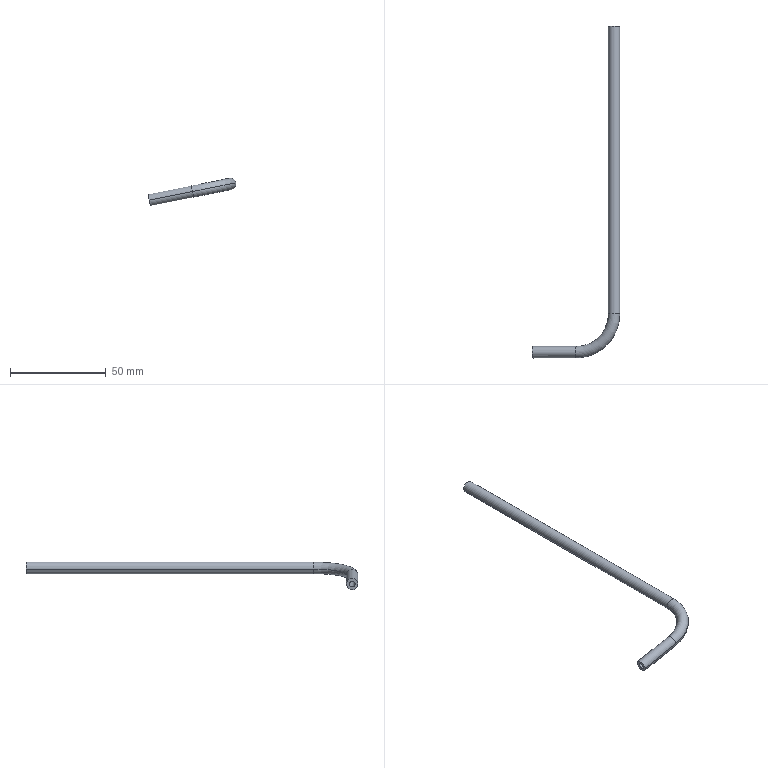Component | SolidWorks | 1-1 | 1 solid | 14 faces | box 45.75 x 173 x 14.39 mm | volume 4335 mm3 | cylinder 8 | torus 4 | plane 2 | commonest cylinder face diameters 3 x4 6 x4
build123d program:
from build123d import *

# Parameters (mm, degrees)
SKETCH7_R   = 3
SKETCH7_R_2 = 1.5


with BuildPart() as part:
    # Sweep2: sweep along a path in Sketch1
    with BuildLine(Plane(origin=(0, 0, 0), x_dir=(1, 0, 0), z_dir=(0, 1, 0))) as sweep2_path:
        Line((0, 0), (0, 23))
        ThreePointArc((0, 23), (-5.858, 37.142), (-20, 43))
        Line((-20, 43), (-170, 43))
    # Sketch7 → Sweep2 (sweep)
    with BuildSketch(Plane(origin=(0, 0, 0), x_dir=(-1, 0, 0), z_dir=(0, 0, -1))):
        Circle(SKETCH7_R)
        Circle(SKETCH7_R_2, mode=Mode.SUBTRACT)
    sweep(path=sweep2_path.line)


solid = part.part

# Placed as in the assembly
solid = solid.moved(Location((80.401, -319.2, 16.115), (-180, -78.666, 90)))
STEP:
#1=CARTESIAN_POINT('',(4.053,-12.508,0.8124));
#2=VERTEX_POINT('',#1);
#3=CARTESIAN_POINT('',(4.053,-12.626,0.8124));
#4=VERTEX_POINT('',#3);
#5=CARTESIAN_POINT('',(4.053,-12.567,0.8124));
#6=DIRECTION('',(-0.9805,-0.,-0.1965));
#7=DIRECTION('',(0.,1.,0.));
#8=AXIS2_PLACEMENT_3D('',#5,#6,#7);
#9=CIRCLE('',#8,0.05906);
#10=EDGE_CURVE('',#2,#4,#9,.T.);
#11=ORIENTED_EDGE('',*,*,#10,.T.);
#12=CARTESIAN_POINT('',(4.883,-11.78,0.9787));
#13=VERTEX_POINT('',#12);
#14=CARTESIAN_POINT('',(4.053,-11.78,0.8124));
#15=DIRECTION('',(-0.1965,-0.,0.9805));
#16=DIRECTION('',(0.9805,0.,0.1965));
#17=AXIS2_PLACEMENT_3D('',#14,#15,#16);
#18=CIRCLE('',#17,0.8465);
#19=EDGE_CURVE('',#4,#13,#18,.T.);
#20=ORIENTED_EDGE('',*,*,#19,.T.);
#21=CARTESIAN_POINT('',(4.767,-11.78,0.9555));
#22=VERTEX_POINT('',#21);
#23=CARTESIAN_POINT('',(4.825,-11.78,0.9671));
#24=DIRECTION('',(0.,-1.,-0.));
#25=DIRECTION('',(-0.9805,0.,-0.1965));
#26=AXIS2_PLACEMENT_3D('',#23,#24,#25);
#27=CIRCLE('',#26,0.05906);
#28=EDGE_CURVE('',#22,#13,#27,.T.);
#29=ORIENTED_EDGE('',*,*,#28,.F.);
#30=CARTESIAN_POINT('',(4.053,-11.78,0.8124));
#31=DIRECTION('',(-0.1965,-0.,0.9805));
#32=DIRECTION('',(0.9805,0.,0.1965));
#33=AXIS2_PLACEMENT_3D('',#30,#31,#32);
#34=CIRCLE('',#33,0.7283);
#35=EDGE_CURVE('',#2,#22,#34,.T.);
#36=ORIENTED_EDGE('',*,*,#35,.F.);
#37=EDGE_LOOP('',(#11,#20,#29,#36));
#38=FACE_OUTER_BOUND('',#37,.T.);
#39=CARTESIAN_POINT('',(4.053,-11.78,0.8124));
#40=DIRECTION('',(-0.1965,-0.,0.9805));
#41=DIRECTION('',(-0.9805,-0.,-0.1965));
#42=AXIS2_PLACEMENT_3D('',#39,#40,#41);
#43=TOROIDAL_SURFACE('',#42,0.7874,0.05906);
#44=ADVANCED_FACE('',(#38),#43,.F.);
#45=CARTESIAN_POINT('',(4.053,-12.449,0.8124));
#46=VERTEX_POINT('',#45);
#47=CARTESIAN_POINT('',(4.053,-12.685,0.8124));
#48=VERTEX_POINT('',#47);
#49=CARTESIAN_POINT('',(4.053,-12.567,0.8124));
#50=DIRECTION('',(0.9805,0.,0.1965));
#51=DIRECTION('',(0.,1.,0.));
#52=AXIS2_PLACEMENT_3D('',#49,#50,#51);
#53=CIRCLE('',#52,0.1181);
#54=EDGE_CURVE('',#46,#48,#53,.T.);
#55=ORIENTED_EDGE('',*,*,#54,.T.);
#56=CARTESIAN_POINT('',(4.941,-11.78,0.9903));
#57=VERTEX_POINT('',#56);
#58=CARTESIAN_POINT('',(4.053,-11.78,0.8124));
#59=DIRECTION('',(-0.1965,-0.,0.9805));
#60=DIRECTION('',(0.9805,0.,0.1965));
#61=AXIS2_PLACEMENT_3D('',#58,#59,#60);
#62=CIRCLE('',#61,0.9055);
#63=EDGE_CURVE('',#48,#57,#62,.T.);
#64=ORIENTED_EDGE('',*,*,#63,.T.);
#65=CARTESIAN_POINT('',(4.709,-11.78,0.9439));
#66=VERTEX_POINT('',#65);
#67=CARTESIAN_POINT('',(4.825,-11.78,0.9671));
#68=DIRECTION('',(-0.,1.,0.));
#69=DIRECTION('',(-0.9805,0.,-0.1965));
#70=AXIS2_PLACEMENT_3D('',#67,#68,#69);
#71=CIRCLE('',#70,0.1181);
#72=EDGE_CURVE('',#66,#57,#71,.T.);
#73=ORIENTED_EDGE('',*,*,#72,.F.);
#74=CARTESIAN_POINT('',(4.053,-11.78,0.8124));
#75=DIRECTION('',(-0.1965,-0.,0.9805));
#76=DIRECTION('',(0.9805,0.,0.1965));
#77=AXIS2_PLACEMENT_3D('',#74,#75,#76);
#78=CIRCLE('',#77,0.6693);
#79=EDGE_CURVE('',#46,#66,#78,.T.);
#80=ORIENTED_EDGE('',*,*,#79,.F.);
#81=EDGE_LOOP('',(#55,#64,#73,#80));
#82=FACE_OUTER_BOUND('',#81,.T.);
#83=CARTESIAN_POINT('',(4.053,-11.78,0.8124));
#84=DIRECTION('',(-0.1965,-0.,0.9805));
#85=DIRECTION('',(-0.9805,0.,-0.1965));
#86=AXIS2_PLACEMENT_3D('',#83,#84,#85);
#87=TOROIDAL_SURFACE('',#86,0.7874,0.1181);
#88=ADVANCED_FACE('',(#82),#87,.T.);
#89=ORIENTED_EDGE('',*,*,#28,.T.);
#90=CARTESIAN_POINT('',(4.883,-5.874,0.9787));
#91=VERTEX_POINT('',#90);
#92=CARTESIAN_POINT('',(4.883,-11.78,0.9787));
#93=DIRECTION('',(-0.,1.,0.));
#94=VECTOR('',#93,39.37);
#95=LINE('',#92,#94);
#96=EDGE_CURVE('',#13,#91,#95,.T.);
#97=ORIENTED_EDGE('',*,*,#96,.T.);
#98=CARTESIAN_POINT('',(4.767,-5.874,0.9555));
#99=VERTEX_POINT('',#98);
#100=CARTESIAN_POINT('',(4.825,-5.874,0.9671));
#101=DIRECTION('',(0.,-1.,-0.));
#102=DIRECTION('',(-0.9805,0.,-0.1965));
#103=AXIS2_PLACEMENT_3D('',#100,#101,#102);
#104=CIRCLE('',#103,0.05906);
#105=EDGE_CURVE('',#99,#91,#104,.T.);
#106=ORIENTED_EDGE('',*,*,#105,.F.);
#107=CARTESIAN_POINT('',(4.767,-11.78,0.9555));
#108=DIRECTION('',(-0.,1.,0.));
#109=VECTOR('',#108,39.37);
#110=LINE('',#107,#109);
#111=EDGE_CURVE('',#22,#99,#110,.T.);
#112=ORIENTED_EDGE('',*,*,#111,.F.);
#113=EDGE_LOOP('',(#89,#97,#106,#112));
#114=FACE_OUTER_BOUND('',#113,.T.);
#115=CARTESIAN_POINT('',(4.825,-11.78,0.9671));
#116=DIRECTION('',(-0.,1.,0.));
#117=DIRECTION('',(-0.9805,0.,-0.1965));
#118=AXIS2_PLACEMENT_3D('',#115,#116,#117);
#119=CYLINDRICAL_SURFACE('',#118,0.05906);
#120=ADVANCED_FACE('',(#114),#119,.F.);
#121=CARTESIAN_POINT('',(3.165,-12.508,0.6344));
#122=VERTEX_POINT('',#121);
#123=CARTESIAN_POINT('',(3.165,-12.626,0.6344));
#124=VERTEX_POINT('',#123);
#125=CARTESIAN_POINT('',(3.165,-12.567,0.6344));
#126=DIRECTION('',(-0.9805,-0.,-0.1965));
#127=DIRECTION('',(0.,1.,0.));
#128=AXIS2_PLACEMENT_3D('',#125,#126,#127);
#129=CIRCLE('',#128,0.05906);
#130=EDGE_CURVE('',#122,#124,#129,.T.);
#131=ORIENTED_EDGE('',*,*,#130,.T.);
#132=CARTESIAN_POINT('',(3.165,-12.626,0.6344));
#133=DIRECTION('',(0.9805,0.,0.1965));
#134=VECTOR('',#133,39.37);
#135=LINE('',#132,#134);
#136=EDGE_CURVE('',#124,#4,#135,.T.);
#137=ORIENTED_EDGE('',*,*,#136,.T.);
#138=ORIENTED_EDGE('',*,*,#10,.F.);
#139=CARTESIAN_POINT('',(3.165,-12.508,0.6344));
#140=DIRECTION('',(0.9805,0.,0.1965));
#141=VECTOR('',#140,39.37);
#142=LINE('',#139,#141);
#143=EDGE_CURVE('',#122,#2,#142,.T.);
#144=ORIENTED_EDGE('',*,*,#143,.F.);
#145=EDGE_LOOP('',(#131,#137,#138,#144));
#146=FACE_OUTER_BOUND('',#145,.T.);
#147=CARTESIAN_POINT('',(3.165,-12.567,0.6344));
#148=DIRECTION('',(0.9805,0.,0.1965));
#149=DIRECTION('',(0.,1.,0.));
#150=AXIS2_PLACEMENT_3D('',#147,#148,#149);
#151=CYLINDRICAL_SURFACE('',#150,0.05906);
#152=ADVANCED_FACE('',(#146),#151,.F.);
#153=ORIENTED_EDGE('',*,*,#72,.T.);
#154=CARTESIAN_POINT('',(4.941,-5.874,0.9903));
#155=VERTEX_POINT('',#154);
#156=CARTESIAN_POINT('',(4.941,-11.78,0.9903));
#157=DIRECTION('',(-0.,1.,0.));
#158=VECTOR('',#157,39.37);
#159=LINE('',#156,#158);
#160=EDGE_CURVE('',#57,#155,#159,.T.);
#161=ORIENTED_EDGE('',*,*,#160,.T.);
#162=CARTESIAN_POINT('',(4.709,-5.874,0.9439));
#163=VERTEX_POINT('',#162);
#164=CARTESIAN_POINT('',(4.825,-5.874,0.9671));
#165=DIRECTION('',(-0.,1.,0.));
#166=DIRECTION('',(-0.9805,0.,-0.1965));
#167=AXIS2_PLACEMENT_3D('',#164,#165,#166);
#168=CIRCLE('',#167,0.1181);
#169=EDGE_CURVE('',#163,#155,#168,.T.);
#170=ORIENTED_EDGE('',*,*,#169,.F.);
#171=CARTESIAN_POINT('',(4.709,-11.78,0.9439));
#172=DIRECTION('',(-0.,1.,0.));
#173=VECTOR('',#172,39.37);
#174=LINE('',#171,#173);
#175=EDGE_CURVE('',#66,#163,#174,.T.);
#176=ORIENTED_EDGE('',*,*,#175,.F.);
#177=EDGE_LOOP('',(#153,#161,#170,#176));
#178=FACE_OUTER_BOUND('',#177,.T.);
#179=CARTESIAN_POINT('',(4.825,-11.78,0.9671));
#180=DIRECTION('',(-0.,1.,0.));
#181=DIRECTION('',(-0.9805,0.,-0.1965));
#182=AXIS2_PLACEMENT_3D('',#179,#180,#181);
#183=CYLINDRICAL_SURFACE('',#182,0.1181);
#184=ADVANCED_FACE('',(#178),#183,.T.);
#185=CARTESIAN_POINT('',(3.165,-12.449,0.6344));
#186=VERTEX_POINT('',#185);
#187=CARTESIAN_POINT('',(3.165,-12.685,0.6344));
#188=VERTEX_POINT('',#187);
#189=CARTESIAN_POINT('',(3.165,-12.567,0.6344));
#190=DIRECTION('',(0.9805,0.,0.1965));
#191=DIRECTION('',(0.,1.,0.));
#192=AXIS2_PLACEMENT_3D('',#189,#190,#191);
#193=CIRCLE('',#192,0.1181);
#194=EDGE_CURVE('',#186,#188,#193,.T.);
#195=ORIENTED_EDGE('',*,*,#194,.T.);
#196=CARTESIAN_POINT('',(3.165,-12.685,0.6344));
#197=DIRECTION('',(0.9805,0.,0.1965));
#198=VECTOR('',#197,39.37);
#199=LINE('',#196,#198);
#200=EDGE_CURVE('',#188,#48,#199,.T.);
#201=ORIENTED_EDGE('',*,*,#200,.T.);
#202=ORIENTED_EDGE('',*,*,#54,.F.);
#203=CARTESIAN_POINT('',(3.165,-12.449,0.6344));
#204=DIRECTION('',(0.9805,0.,0.1965));
#205=VECTOR('',#204,39.37);
#206=LINE('',#203,#205);
#207=EDGE_CURVE('',#186,#46,#206,.T.);
#208=ORIENTED_EDGE('',*,*,#207,.F.);
#209=EDGE_LOOP('',(#195,#201,#202,#208));
#210=FACE_OUTER_BOUND('',#209,.T.);
#211=CARTESIAN_POINT('',(3.165,-12.567,0.6344));
#212=DIRECTION('',(0.9805,0.,0.1965));
#213=DIRECTION('',(0.,1.,0.));
#214=AXIS2_PLACEMENT_3D('',#211,#212,#213);
#215=CYLINDRICAL_SURFACE('',#214,0.1181);
#216=ADVANCED_FACE('',(#210),#215,.T.);
#217=ORIENTED_EDGE('',*,*,#96,.F.);
#218=CARTESIAN_POINT('',(4.825,-11.78,0.9671));
#219=DIRECTION('',(0.,-1.,-0.));
#220=DIRECTION('',(-0.9805,0.,-0.1965));
#221=AXIS2_PLACEMENT_3D('',#218,#219,#220);
#222=CIRCLE('',#221,0.05906);
#223=EDGE_CURVE('',#13,#22,#222,.T.);
#224=ORIENTED_EDGE('',*,*,#223,.T.);
#225=ORIENTED_EDGE('',*,*,#111,.T.);
#226=CARTESIAN_POINT('',(4.825,-5.874,0.9671));
#227=DIRECTION('',(0.,-1.,-0.));
#228=DIRECTION('',(-0.9805,0.,-0.1965));
#229=AXIS2_PLACEMENT_3D('',#226,#227,#228);
#230=CIRCLE('',#229,0.05906);
#231=EDGE_CURVE('',#91,#99,#230,.T.);
#232=ORIENTED_EDGE('',*,*,#231,.F.);
#233=EDGE_LOOP('',(#217,#224,#225,#232));
#234=FACE_OUTER_BOUND('',#233,.T.);
#235=CARTESIAN_POINT('',(4.825,-11.78,0.9671));
#236=DIRECTION('',(-0.,1.,0.));
#237=DIRECTION('',(-0.9805,0.,-0.1965));
#238=AXIS2_PLACEMENT_3D('',#235,#236,#237);
#239=CYLINDRICAL_SURFACE('',#238,0.05906);
#240=ADVANCED_FACE('',(#234),#239,.F.);
#241=ORIENTED_EDGE('',*,*,#19,.F.);
#242=CARTESIAN_POINT('',(4.053,-12.567,0.8124));
#243=DIRECTION('',(-0.9805,-0.,-0.1965));
#244=DIRECTION('',(0.,1.,-0.));
#245=AXIS2_PLACEMENT_3D('',#242,#243,#244);
#246=CIRCLE('',#245,0.05906);
#247=EDGE_CURVE('',#4,#2,#246,.T.);
#248=ORIENTED_EDGE('',*,*,#247,.T.);
#249=ORIENTED_EDGE('',*,*,#35,.T.);
#250=ORIENTED_EDGE('',*,*,#223,.F.);
#251=EDGE_LOOP('',(#241,#248,#249,#250));
#252=FACE_OUTER_BOUND('',#251,.T.);
#253=CARTESIAN_POINT('',(4.053,-11.78,0.8124));
#254=DIRECTION('',(-0.1965,-0.,0.9805));
#255=DIRECTION('',(-0.9805,-0.,-0.1965));
#256=AXIS2_PLACEMENT_3D('',#253,#254,#255);
#257=TOROIDAL_SURFACE('',#256,0.7874,0.05906);
#258=ADVANCED_FACE('',(#252),#257,.F.);
#259=ORIENTED_EDGE('',*,*,#136,.F.);
#260=CARTESIAN_POINT('',(3.165,-12.567,0.6344));
#261=DIRECTION('',(-0.9805,-0.,-0.1965));
#262=DIRECTION('',(0.,1.,0.));
#263=AXIS2_PLACEMENT_3D('',#260,#261,#262);
#264=CIRCLE('',#263,0.05906);
#265=EDGE_CURVE('',#124,#122,#264,.T.);
#266=ORIENTED_EDGE('',*,*,#265,.T.);
#267=ORIENTED_EDGE('',*,*,#143,.T.);
#268=ORIENTED_EDGE('',*,*,#247,.F.);
#269=EDGE_LOOP('',(#259,#266,#267,#268));
#270=FACE_OUTER_BOUND('',#269,.T.);
#271=CARTESIAN_POINT('',(3.165,-12.567,0.6344));
#272=DIRECTION('',(0.9805,0.,0.1965));
#273=DIRECTION('',(0.,1.,0.));
#274=AXIS2_PLACEMENT_3D('',#271,#272,#273);
#275=CYLINDRICAL_SURFACE('',#274,0.05906);
#276=ADVANCED_FACE('',(#270),#275,.F.);
#277=ORIENTED_EDGE('',*,*,#105,.T.);
#278=ORIENTED_EDGE('',*,*,#231,.T.);
#279=EDGE_LOOP('',(#277,#278));
#280=FACE_BOUND('',#279,.T.);
#281=ORIENTED_EDGE('',*,*,#169,.T.);
#282=CARTESIAN_POINT('',(4.825,-5.874,0.9671));
#283=DIRECTION('',(-0.,1.,0.));
#284=DIRECTION('',(-0.9805,0.,-0.1965));
#285=AXIS2_PLACEMENT_3D('',#282,#283,#284);
#286=CIRCLE('',#285,0.1181);
#287=EDGE_CURVE('',#155,#163,#286,.T.);
#288=ORIENTED_EDGE('',*,*,#287,.T.);
#289=EDGE_LOOP('',(#281,#288));
#290=FACE_OUTER_BOUND('',#289,.T.);
#291=CARTESIAN_POINT('',(4.825,-5.874,0.9671));
#292=DIRECTION('',(-0.,1.,0.));
#293=DIRECTION('',(-0.9805,-0.,-0.1965));
#294=AXIS2_PLACEMENT_3D('',#291,#292,#293);
#295=PLANE('',#294);
#296=ADVANCED_FACE('',(#280,#290),#295,.T.);
#297=ORIENTED_EDGE('',*,*,#130,.F.);
#298=ORIENTED_EDGE('',*,*,#265,.F.);
#299=EDGE_LOOP('',(#297,#298));
#300=FACE_BOUND('',#299,.T.);
#301=ORIENTED_EDGE('',*,*,#194,.F.);
#302=CARTESIAN_POINT('',(3.165,-12.567,0.6344));
#303=DIRECTION('',(0.9805,0.,0.1965));
#304=DIRECTION('',(0.,1.,0.));
#305=AXIS2_PLACEMENT_3D('',#302,#303,#304);
#306=CIRCLE('',#305,0.1181);
#307=EDGE_CURVE('',#188,#186,#306,.T.);
#308=ORIENTED_EDGE('',*,*,#307,.F.);
#309=EDGE_LOOP('',(#301,#308));
#310=FACE_OUTER_BOUND('',#309,.T.);
#311=CARTESIAN_POINT('',(3.165,-12.567,0.6344));
#312=DIRECTION('',(0.9805,0.,0.1965));
#313=DIRECTION('',(-0.,1.,0.));
#314=AXIS2_PLACEMENT_3D('',#311,#312,#313);
#315=PLANE('',#314);
#316=ADVANCED_FACE('',(#300,#310),#315,.F.);
#317=ORIENTED_EDGE('',*,*,#160,.F.);
#318=CARTESIAN_POINT('',(4.825,-11.78,0.9671));
#319=DIRECTION('',(-0.,1.,0.));
#320=DIRECTION('',(-0.9805,0.,-0.1965));
#321=AXIS2_PLACEMENT_3D('',#318,#319,#320);
#322=CIRCLE('',#321,0.1181);
#323=EDGE_CURVE('',#57,#66,#322,.T.);
#324=ORIENTED_EDGE('',*,*,#323,.T.);
#325=ORIENTED_EDGE('',*,*,#175,.T.);
#326=ORIENTED_EDGE('',*,*,#287,.F.);
#327=EDGE_LOOP('',(#317,#324,#325,#326));
#328=FACE_OUTER_BOUND('',#327,.T.);
#329=CARTESIAN_POINT('',(4.825,-11.78,0.9671));
#330=DIRECTION('',(-0.,1.,0.));
#331=DIRECTION('',(-0.9805,0.,-0.1965));
#332=AXIS2_PLACEMENT_3D('',#329,#330,#331);
#333=CYLINDRICAL_SURFACE('',#332,0.1181);
#334=ADVANCED_FACE('',(#328),#333,.T.);
#335=ORIENTED_EDGE('',*,*,#63,.F.);
#336=CARTESIAN_POINT('',(4.053,-12.567,0.8124));
#337=DIRECTION('',(0.9805,0.,0.1965));
#338=DIRECTION('',(0.,1.,0.));
#339=AXIS2_PLACEMENT_3D('',#336,#337,#338);
#340=CIRCLE('',#339,0.1181);
#341=EDGE_CURVE('',#48,#46,#340,.T.);
#342=ORIENTED_EDGE('',*,*,#341,.T.);
#343=ORIENTED_EDGE('',*,*,#79,.T.);
#344=ORIENTED_EDGE('',*,*,#323,.F.);
#345=EDGE_LOOP('',(#335,#342,#343,#344));
#346=FACE_OUTER_BOUND('',#345,.T.);
#347=CARTESIAN_POINT('',(4.053,-11.78,0.8124));
#348=DIRECTION('',(-0.1965,-0.,0.9805));
#349=DIRECTION('',(-0.9805,0.,-0.1965));
#350=AXIS2_PLACEMENT_3D('',#347,#348,#349);
#351=TOROIDAL_SURFACE('',#350,0.7874,0.1181);
#352=ADVANCED_FACE('',(#346),#351,.T.);
#353=ORIENTED_EDGE('',*,*,#200,.F.);
#354=ORIENTED_EDGE('',*,*,#307,.T.);
#355=ORIENTED_EDGE('',*,*,#207,.T.);
#356=ORIENTED_EDGE('',*,*,#341,.F.);
#357=EDGE_LOOP('',(#353,#354,#355,#356));
#358=FACE_OUTER_BOUND('',#357,.T.);
#359=CARTESIAN_POINT('',(3.165,-12.567,0.6344));
#360=DIRECTION('',(0.9805,0.,0.1965));
#361=DIRECTION('',(0.,1.,0.));
#362=AXIS2_PLACEMENT_3D('',#359,#360,#361);
#363=CYLINDRICAL_SURFACE('',#362,0.1181);
#364=ADVANCED_FACE('',(#358),#363,.T.);
#365=CLOSED_SHELL('',(#44,#88,#120,#152,#184,#216,#240,#258,#276,#296,#316,#334,#352,#364));
#366=MANIFOLD_SOLID_BREP('',#365);
#367=CARTESIAN_POINT('',(0.,0.,0.));
#368=DIRECTION('',(0.,0.,1.));
#369=DIRECTION('',(1.,0.,0.));
#370=AXIS2_PLACEMENT_3D('',#367,#368,#369);
#371=(LENGTH_UNIT()NAMED_UNIT(*)SI_UNIT($,.METRE.));
#372=LENGTH_MEASURE_WITH_UNIT(LENGTH_MEASURE(0.0254),#371);
#373=DIMENSIONAL_EXPONENTS(1.,0.,0.,0.,0.,0.,0.);
#374=(CONVERSION_BASED_UNIT('',#372)LENGTH_UNIT()NAMED_UNIT(#373));
#375=UNCERTAINTY_MEASURE_WITH_UNIT(LENGTH_MEASURE(0.00001),#374,'','');
#376=(NAMED_UNIT(*)PLANE_ANGLE_UNIT()SI_UNIT($,.RADIAN.));
#377=(NAMED_UNIT(*)SI_UNIT($,.STERADIAN.)SOLID_ANGLE_UNIT());
#378=(GEOMETRIC_REPRESENTATION_CONTEXT(3)GLOBAL_UNCERTAINTY_ASSIGNED_CONTEXT((#375))GLOBAL_UNIT_ASSIGNED_CONTEXT((#374,#376,#377))REPRESENTATION_CONTEXT('',''));
#379=ADVANCED_BREP_SHAPE_REPRESENTATION('',(#366,#370),#378);
#380=COLOUR_RGB('',0.7922,0.8196,0.9333);
#381=FILL_AREA_STYLE_COLOUR('',#380);
#382=FILL_AREA_STYLE('',(#381));
#383=SURFACE_STYLE_FILL_AREA(#382);
#384=SURFACE_SIDE_STYLE('',(#383));
#385=SURFACE_STYLE_USAGE(.BOTH.,#384);
#386=PRESENTATION_STYLE_ASSIGNMENT((#385));
#387=STYLED_ITEM('',(#386),#366);
#388=(LENGTH_UNIT()NAMED_UNIT(*)SI_UNIT($,.METRE.));
#389=LENGTH_MEASURE_WITH_UNIT(LENGTH_MEASURE(0.0254),#388);
#390=DIMENSIONAL_EXPONENTS(1.,0.,0.,0.,0.,0.,0.);
#391=(CONVERSION_BASED_UNIT('',#389)LENGTH_UNIT()NAMED_UNIT(#390));
#392=UNCERTAINTY_MEASURE_WITH_UNIT(LENGTH_MEASURE(0.00001),#391,'','');
#393=(NAMED_UNIT(*)PLANE_ANGLE_UNIT()SI_UNIT($,.RADIAN.));
#394=(NAMED_UNIT(*)SI_UNIT($,.STERADIAN.)SOLID_ANGLE_UNIT());
#395=(GEOMETRIC_REPRESENTATION_CONTEXT(3)GLOBAL_UNCERTAINTY_ASSIGNED_CONTEXT((#392))GLOBAL_UNIT_ASSIGNED_CONTEXT((#391,#393,#394))REPRESENTATION_CONTEXT('',''));
#396=MECHANICAL_DESIGN_GEOMETRIC_PRESENTATION_REPRESENTATION('',(#387),#395);
#397=PRESENTATION_LAYER_ASSIGNMENT('','',(#387));